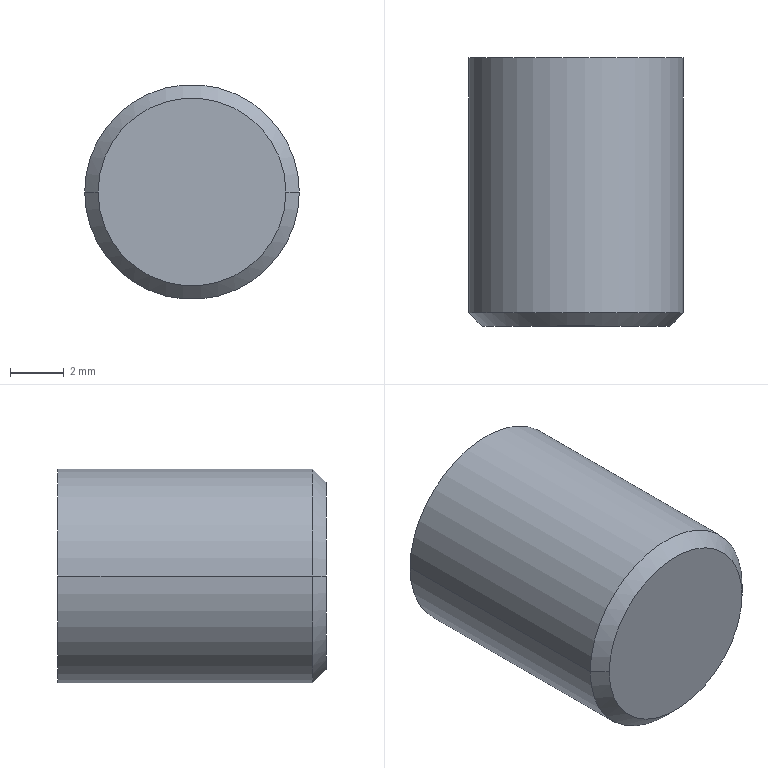Component | SolidWorks | BSH3-03-39Pin-1 | 1 solid | 6 faces | box 8 x 10 x 8 mm | volume 500 mm3 | cone 2 | cylinder 2 | plane 2 | commonest cylinder face diameters 8 x2
build123d program:
from build123d import *

# Parameters (mm, degrees)
SKETCH1_R      = 4
EXTRUDE1_DEPTH = 10
CHAMFER1_SIZE  = 0.5


with BuildPart() as part:
    # Sketch1 → Extrude1 (new body)
    with BuildSketch(Plane.XY):
        Circle(SKETCH1_R)
    extrude(amount=EXTRUDE1_DEPTH)

    # Chamfer1
    chamfer1_edges = [part.edges().sort_by_distance(p)[0] for p in [
        (-4, 0, 0),
    ]]
    chamfer(chamfer1_edges, length=CHAMFER1_SIZE)


solid = part.part

# Placed as in the assembly
solid = solid.moved(Location((88.129, 18.012, -20.589), (-90, 0, 0)))
STEP:
#1=COLOUR_RGB('',0.7922,0.8196,0.9333);
#2=FILL_AREA_STYLE_COLOUR('',#1);
#3=FILL_AREA_STYLE('',(#2));
#4=SURFACE_STYLE_FILL_AREA(#3);
#5=SURFACE_SIDE_STYLE('',(#4));
#6=SURFACE_STYLE_USAGE(.BOTH.,#5);
#7=PRESENTATION_STYLE_ASSIGNMENT((#6));
#8=CARTESIAN_POINT('',(3.332,0.7091,-0.8106));
#9=VERTEX_POINT('',#8);
#10=CARTESIAN_POINT('',(3.607,0.7091,-0.8106));
#11=VERTEX_POINT('',#10);
#12=CARTESIAN_POINT('',(3.47,0.7091,-0.8106));
#13=DIRECTION('',(0.,-1.,0.));
#14=DIRECTION('',(1.,0.,0.));
#15=AXIS2_PLACEMENT_3D('',#12,#13,#14);
#16=CIRCLE('',#15,0.1378);
#17=EDGE_CURVE('',#9,#11,#16,.T.);
#18=ORIENTED_EDGE('',*,*,#17,.F.);
#19=CARTESIAN_POINT('',(3.312,0.7288,-0.8106));
#20=VERTEX_POINT('',#19);
#21=CARTESIAN_POINT('',(3.312,0.7288,-0.8106));
#22=DIRECTION('',(-0.7071,0.7071,-0.));
#23=VECTOR('',#22,39.37);
#24=LINE('',#21,#23);
#25=EDGE_CURVE('',#9,#20,#24,.T.);
#26=ORIENTED_EDGE('',*,*,#25,.T.);
#27=CARTESIAN_POINT('',(3.627,0.7288,-0.8106));
#28=VERTEX_POINT('',#27);
#29=CARTESIAN_POINT('',(3.47,0.7288,-0.8106));
#30=DIRECTION('',(-0.,1.,0.));
#31=DIRECTION('',(1.,0.,0.));
#32=AXIS2_PLACEMENT_3D('',#29,#30,#31);
#33=CIRCLE('',#32,0.1575);
#34=EDGE_CURVE('',#28,#20,#33,.T.);
#35=ORIENTED_EDGE('',*,*,#34,.F.);
#36=CARTESIAN_POINT('',(3.627,0.7288,-0.8106));
#37=DIRECTION('',(0.7071,0.7071,0.));
#38=VECTOR('',#37,39.37);
#39=LINE('',#36,#38);
#40=EDGE_CURVE('',#11,#28,#39,.T.);
#41=ORIENTED_EDGE('',*,*,#40,.F.);
#42=EDGE_LOOP('',(#18,#26,#35,#41));
#43=FACE_OUTER_BOUND('',#42,.T.);
#44=CARTESIAN_POINT('',(3.47,0.7288,-0.8106));
#45=DIRECTION('',(-0.,1.,0.));
#46=DIRECTION('',(1.,0.,0.));
#47=AXIS2_PLACEMENT_3D('',#44,#45,#46);
#48=CONICAL_SURFACE('',#47,0.1575,0.7854);
#49=ADVANCED_FACE('',(#43),#48,.T.);
#50=CARTESIAN_POINT('',(3.627,1.103,-0.8106));
#51=VERTEX_POINT('',#50);
#52=CARTESIAN_POINT('',(3.312,1.103,-0.8106));
#53=VERTEX_POINT('',#52);
#54=CARTESIAN_POINT('',(3.47,1.103,-0.8106));
#55=DIRECTION('',(-0.,1.,0.));
#56=DIRECTION('',(1.,0.,0.));
#57=AXIS2_PLACEMENT_3D('',#54,#55,#56);
#58=CIRCLE('',#57,0.1575);
#59=EDGE_CURVE('',#51,#53,#58,.T.);
#60=ORIENTED_EDGE('',*,*,#59,.F.);
#61=CARTESIAN_POINT('',(3.627,1.103,-0.8106));
#62=DIRECTION('',(0.,-1.,0.));
#63=VECTOR('',#62,39.37);
#64=LINE('',#61,#63);
#65=EDGE_CURVE('',#51,#28,#64,.T.);
#66=ORIENTED_EDGE('',*,*,#65,.T.);
#67=ORIENTED_EDGE('',*,*,#34,.T.);
#68=CARTESIAN_POINT('',(3.312,1.103,-0.8106));
#69=DIRECTION('',(0.,-1.,0.));
#70=VECTOR('',#69,39.37);
#71=LINE('',#68,#70);
#72=EDGE_CURVE('',#53,#20,#71,.T.);
#73=ORIENTED_EDGE('',*,*,#72,.F.);
#74=EDGE_LOOP('',(#60,#66,#67,#73));
#75=FACE_OUTER_BOUND('',#74,.T.);
#76=CARTESIAN_POINT('',(3.47,1.103,-0.8106));
#77=DIRECTION('',(0.,-1.,0.));
#78=DIRECTION('',(-1.,0.,0.));
#79=AXIS2_PLACEMENT_3D('',#76,#77,#78);
#80=CYLINDRICAL_SURFACE('',#79,0.1575);
#81=ADVANCED_FACE('',(#75),#80,.T.);
#82=ORIENTED_EDGE('',*,*,#65,.F.);
#83=CARTESIAN_POINT('',(3.47,1.103,-0.8106));
#84=DIRECTION('',(-0.,1.,0.));
#85=DIRECTION('',(1.,0.,0.));
#86=AXIS2_PLACEMENT_3D('',#83,#84,#85);
#87=CIRCLE('',#86,0.1575);
#88=EDGE_CURVE('',#53,#51,#87,.T.);
#89=ORIENTED_EDGE('',*,*,#88,.F.);
#90=ORIENTED_EDGE('',*,*,#72,.T.);
#91=CARTESIAN_POINT('',(3.47,0.7288,-0.8106));
#92=DIRECTION('',(-0.,1.,0.));
#93=DIRECTION('',(1.,0.,0.));
#94=AXIS2_PLACEMENT_3D('',#91,#92,#93);
#95=CIRCLE('',#94,0.1575);
#96=EDGE_CURVE('',#20,#28,#95,.T.);
#97=ORIENTED_EDGE('',*,*,#96,.T.);
#98=EDGE_LOOP('',(#82,#89,#90,#97));
#99=FACE_OUTER_BOUND('',#98,.T.);
#100=CARTESIAN_POINT('',(3.47,1.103,-0.8106));
#101=DIRECTION('',(0.,-1.,0.));
#102=DIRECTION('',(-1.,0.,0.));
#103=AXIS2_PLACEMENT_3D('',#100,#101,#102);
#104=CYLINDRICAL_SURFACE('',#103,0.1575);
#105=ADVANCED_FACE('',(#99),#104,.T.);
#106=ORIENTED_EDGE('',*,*,#88,.T.);
#107=ORIENTED_EDGE('',*,*,#59,.T.);
#108=EDGE_LOOP('',(#106,#107));
#109=FACE_OUTER_BOUND('',#108,.T.);
#110=CARTESIAN_POINT('',(3.47,1.103,-0.8106));
#111=DIRECTION('',(-0.,1.,0.));
#112=DIRECTION('',(1.,0.,0.));
#113=AXIS2_PLACEMENT_3D('',#110,#111,#112);
#114=PLANE('',#113);
#115=ADVANCED_FACE('',(#109),#114,.T.);
#116=CARTESIAN_POINT('',(3.47,0.7091,-0.8106));
#117=DIRECTION('',(0.,-1.,0.));
#118=DIRECTION('',(1.,0.,0.));
#119=AXIS2_PLACEMENT_3D('',#116,#117,#118);
#120=CIRCLE('',#119,0.1378);
#121=EDGE_CURVE('',#11,#9,#120,.T.);
#122=ORIENTED_EDGE('',*,*,#121,.T.);
#123=ORIENTED_EDGE('',*,*,#17,.T.);
#124=EDGE_LOOP('',(#122,#123));
#125=FACE_OUTER_BOUND('',#124,.T.);
#126=CARTESIAN_POINT('',(3.47,0.7091,-0.8106));
#127=DIRECTION('',(-0.,1.,0.));
#128=DIRECTION('',(1.,0.,0.));
#129=AXIS2_PLACEMENT_3D('',#126,#127,#128);
#130=PLANE('',#129);
#131=ADVANCED_FACE('',(#125),#130,.F.);
#132=ORIENTED_EDGE('',*,*,#25,.F.);
#133=ORIENTED_EDGE('',*,*,#121,.F.);
#134=ORIENTED_EDGE('',*,*,#40,.T.);
#135=ORIENTED_EDGE('',*,*,#96,.F.);
#136=EDGE_LOOP('',(#132,#133,#134,#135));
#137=FACE_OUTER_BOUND('',#136,.T.);
#138=CARTESIAN_POINT('',(3.47,0.7288,-0.8106));
#139=DIRECTION('',(-0.,1.,0.));
#140=DIRECTION('',(1.,0.,0.));
#141=AXIS2_PLACEMENT_3D('',#138,#139,#140);
#142=CONICAL_SURFACE('',#141,0.1575,0.7854);
#143=ADVANCED_FACE('',(#137),#142,.T.);
#144=CLOSED_SHELL('',(#49,#81,#105,#115,#131,#143));
#145=MANIFOLD_SOLID_BREP('',#144);
#146=STYLED_ITEM('',(#7),#145);
#147=(LENGTH_UNIT()NAMED_UNIT(*)SI_UNIT($,.METRE.));
#148=LENGTH_MEASURE_WITH_UNIT(LENGTH_MEASURE(0.0254),#147);
#149=DIMENSIONAL_EXPONENTS(1.,0.,0.,0.,0.,0.,0.);
#150=(CONVERSION_BASED_UNIT('',#148)LENGTH_UNIT()NAMED_UNIT(#149));
#151=UNCERTAINTY_MEASURE_WITH_UNIT(LENGTH_MEASURE(0.00001),#150,'','');
#152=(NAMED_UNIT(*)PLANE_ANGLE_UNIT()SI_UNIT($,.RADIAN.));
#153=(NAMED_UNIT(*)SI_UNIT($,.STERADIAN.)SOLID_ANGLE_UNIT());
#154=(GEOMETRIC_REPRESENTATION_CONTEXT(3)GLOBAL_UNCERTAINTY_ASSIGNED_CONTEXT((#151))GLOBAL_UNIT_ASSIGNED_CONTEXT((#150,#152,#153))REPRESENTATION_CONTEXT('',''));
#155=MECHANICAL_DESIGN_GEOMETRIC_PRESENTATION_REPRESENTATION('',(#146),#154);
#156=PRESENTATION_LAYER_ASSIGNMENT('','',(#146));
#157=CARTESIAN_POINT('',(0.,0.,0.));
#158=DIRECTION('',(0.,0.,1.));
#159=DIRECTION('',(1.,0.,0.));
#160=AXIS2_PLACEMENT_3D('',#157,#158,#159);
#161=(LENGTH_UNIT()NAMED_UNIT(*)SI_UNIT($,.METRE.));
#162=LENGTH_MEASURE_WITH_UNIT(LENGTH_MEASURE(0.0254),#161);
#163=DIMENSIONAL_EXPONENTS(1.,0.,0.,0.,0.,0.,0.);
#164=(CONVERSION_BASED_UNIT('',#162)LENGTH_UNIT()NAMED_UNIT(#163));
#165=UNCERTAINTY_MEASURE_WITH_UNIT(LENGTH_MEASURE(0.00001),#164,'','');
#166=(NAMED_UNIT(*)PLANE_ANGLE_UNIT()SI_UNIT($,.RADIAN.));
#167=(NAMED_UNIT(*)SI_UNIT($,.STERADIAN.)SOLID_ANGLE_UNIT());
#168=(GEOMETRIC_REPRESENTATION_CONTEXT(3)GLOBAL_UNCERTAINTY_ASSIGNED_CONTEXT((#165))GLOBAL_UNIT_ASSIGNED_CONTEXT((#164,#166,#167))REPRESENTATION_CONTEXT('',''));
#169=ADVANCED_BREP_SHAPE_REPRESENTATION('',(#145,#160),#168);